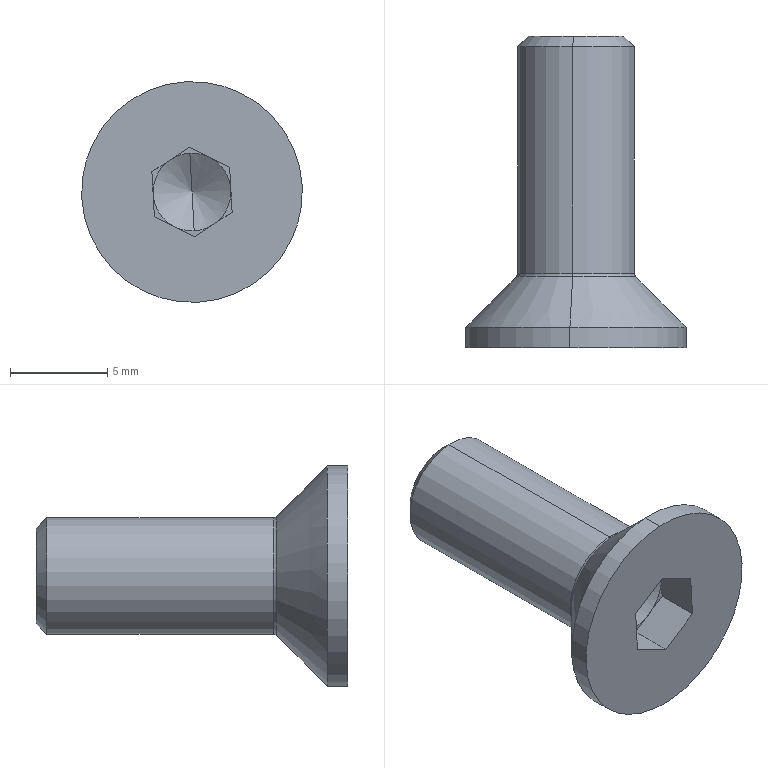Component | SolidWorks | hexagon socket countersunk head screws gb-1 | 1 solid | 26 faces | volume 578 mm3 | plane 14 | cone 6 | cylinder 4 | torus 2 | commonest cylinder face diameters 11.34 x2 6 x2